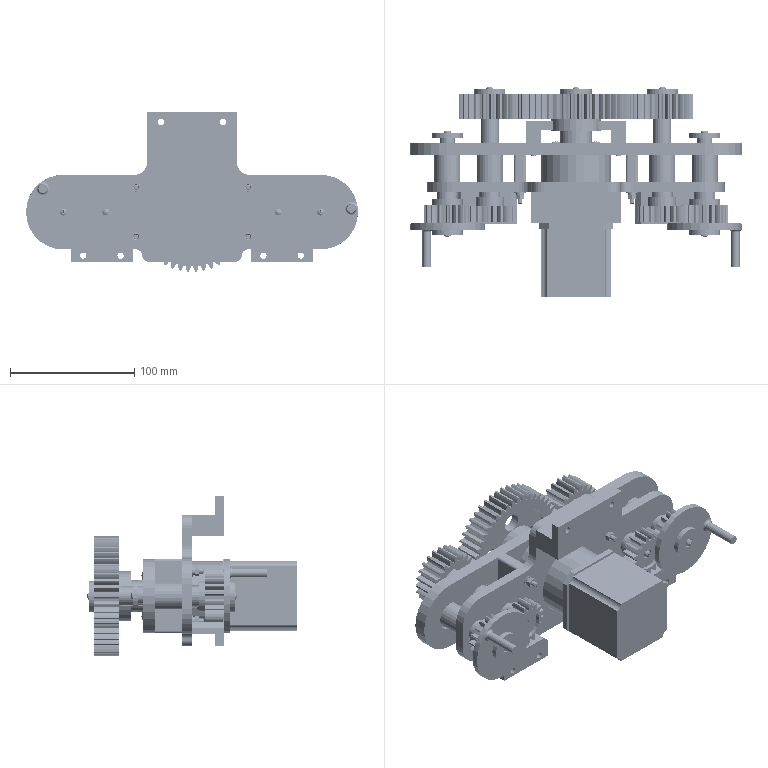Assembly | SolidWorks | mm | 113 component files | 113 solids | 4021 faces | box 266.76 x 168.69 x 128.09 mm | volume 977841 mm3 | cylinder 1324 | torus 964 | plane 785 | sphere 578 | cone 186 | spline 184 | commonest cylinder face diameters 13.6 x152 5 x65 4 x60 15 x54 87 x47 3 x46 96 x46 50 x46
Bill of materials:
23-ToothGear | 2 |  | Spur gear with straight teeth (roughly 24 teeth) and a central round bore with one rectangular keyway notch; a raised annular hub or boss sits on one face.
46-ToothGear | 1 |  | Spur gear with fine straight teeth (roughly 44 teeth), a central bore with a keyway notch, and four evenly spaced circular lightening or through holes around the bore; a short hub is visible on one face.
BearingHousing | 1 | A-Glass Fiber | Bracket with a central thick annular ring and two rectangular arms on opposite sides. Each arm steps down into an offset block, and each block has a small through hole running along the arm direction.
CrankshaftNo.1 | 2 | 5154-O, Bar (SS) | Stepped round shaft with several coaxial diameter sections. The largest section is near the middle, and both ends are smaller. One end section has a lengthwise keyway slot, and the end faces show small conical center holes.
Rolling bearings 61803 GB 276-94 | 4 |  | Ball-bearing-like ring set: thin flat outer ring and inner ring, with one row of spherical balls (about 30) in the annular gap; there are faint, irregular features near the inner ring that could be a cage or mesh artifacts.
Rolling bearings 61802 GB 276-94 | 4 |  | Ball-bearing-like ring set: flat outer and inner rings with one row of spherical balls (about 28) in the annular gap; open faces with no visible cage or shield.
NewCrank | 2 | AISI 1045 Steel, Cold Drawn | Flat circular disc with a central bore that has a keyway notch. A single cylindrical pin projects perpendicular to the disc face near the outer edge, with a fillet where it meets the disc.
GB - Spur gear 2M 17T 20PA 15FW ---S17B25H20L15.0S1 | 2 |  | Spur-gear-like body with about 17 straight teeth cut parallel to the axis, a round central bore with a rectangular keyway-like notch, and a smaller-diameter cylindrical hub boss on one face.
Rolling bearings 61804 GB 276-94 | 2 |  | Ball-bearing-like ring set: flat outer and inner rings with one row of spherical balls (about 28) in the annular gap; open faces with no visible cage or shield.
DialAxisNo.3 | 1 |  | Stepped cylindrical shaft/sleeve with a larger collar between two medium-diameter sections and a smaller-diameter spigot at one end. The larger end has an internal bore with a keyway notch, and the small spigot has an external lengthwise keyway slot.
EndCap4mm | 9 | 5454-O | Plain flat circular disc with a small central through hole and uniform thickness.
GB 93-87-3 | 9 |  | Split ring with a rectangular cross-section and a single narrow radial gap through the ring. It looks like a split or spring-type washer.
GB 93-87-4 | 10 |  | Split ring with a rectangular cross-section and a single narrow radial gap. It looks like a split or spring-type washer.
GB_T1096-1979PlainParallelKeyC-type5_12 | 2 |  | Rectangular-section bar with one end fully rounded and the other end square. All long edges are lightly rounded. It looks like a parallel key.
GB_T1096-1979PlainParallelKeyC-type5_18 | 3 |  | Rectangular-section bar with one rounded end and one square-cut end, and lightly rounded long edges. It looks like a parallel key.
GB_T1096-1979PlainParallelKeyC-type5_25 | 1 |  | Long rectangular-section bar with a rounded end visible at one end, a square-cut opposite end, and small edge rounds. It looks like a parallel key.
GB_T1096-1979PlainParallelKeyC-type5_25 | 2 |  | Straight bar with a near-square cross-section and rounded longitudinal edges. One end is flat and square-cut; the other end is fully rounded (semicircular) in one view. The shape looks like a parallel key.
GB_T6170-2000Type1HexNutGradeAAndBM4 | 4 |  | Hexagonal nut-like prism with a central through bore and chamfered corners on both faces.
GB_T818-2000PhillipsPanHeadScrewM3_12 | 9 |  | Fastener-like pin with a slotted domed head and a smooth cylindrical shank. The shank has a short reduced-diameter neck under the head and a chamfered tip.
GB_T818-2000PhillipsPanHeadScrewM4_12 | 4 |  | Slotted domed-head pin or screw-like part with a short smooth shank, a reduced neck under the head and a chamfered tip. Shorter and stubbier than similar parts in this set.
GB_T818-2000PhillipsPanHeadScrewM4_25 | 2 |  | Long, slender slotted domed-head pin or screw-like part with a smooth shank, a reduced neck under the head and a chamfered tip.
GB_T818-2000PhillipsPanHeadScrewM4_45 | 4 |  | Very long, slender slotted domed-head pin or screw-like part with a smooth shank, a small neck under the head and a chamfered tip.
GB_T95-2002FlatWasherCClass4x0.8 | 10 |  | Flat annular washer-like ring with a central circular hole and plain flat faces.
GB_T95-2002FlatWasherGradeC3_0.5 | 9 |  | Flat annular washer-like ring with a central circular hole. It looks slightly thinner than unnamed part.
GB823-88PhillipsSmallPanHeadScrewM5_14 | 2 |  | Short slotted domed-head pin or screw-like part. It has a relatively large head, a smooth shank, a reduced neck under the head and a chamfered tip.
GearIntermediateAxis | 2 | 5154-O, Bar (SS) | Stepped cylindrical shaft. It has a larger central collar, several smaller diameter steps toward each end, a keyway-like slot near each end and a small axial center hole in one end face.
GenevaWheelUpperGear(45Steel) | 2 |  | Spur-gear-like toothed wheel with a cylindrical hub on one side and a central bore with one rectangular keyway notch.
LatestLowerBaseFrame | 1 | 6061 Alloy | Thin flat plate with a cross or T-like outline and rounded corners. It has one large central hole, four medium round holes in line along the long axis, and several small holes.
LatestStepperMotor | 1 | AISI 1045 Steel, Cold Drawn | Simplified housing-like body. A square block with chamfered corners joins through a thin flange or collar to a cylindrical section, and a small stepped cylindrical shaft projects from the far end.
LegSupport | 2 |  | Prismatic block with an L-shaped cross-section (a full-width top portion over a narrower lower leg along one side), angled chamfers on the top edges at both short ends, and two round through holes in the long front face near each end.
LegSupport2 | 1 |  | Long rectangular bar with an L-shaped cross-section (a rabbet or step cut along one long top edge for the full length) and two round through holes in the large side face near the ends.
Support | 2 |  | Rectangular block or spacer bar with rounded long edges, and two round through holes passing through its narrow dimension near each end.
UpperBracket | 1 | 6061-T6 (SS) | Thin flat plate with a slot-shaped (obround) outline and fully rounded ends. It has a large central hole, four medium holes in line along the long axis (two near each end), and ten small holes grouped symmetrically around the center.
Mates:
1. concentric | LatestLowerBaseFrame-1 face at (-121.534, 78.266, -110.507) dir (0, 1, 0) r 2.5 | LegSupport2-1 face at (-121.534, 78.266, -110.507) dir (0, 1, 0) r 2.5
2. concentric | LatestLowerBaseFrame-1 face at (-71.534, 78.266, -110.507) dir (0, 1, 0) r 2.5 | LegSupport2-1 face at (-71.534, 78.266, -110.507) dir (0, 1, 0) r 2.5
3. coincident | LatestLowerBaseFrame-1 face at (-96.534, 78.266, -166.507) dir (0, -1, 0) | LegSupport2-1 face at (-96.534, 78.266, -102.347) dir (0, 1, 0)
4. concentric | LatestLowerBaseFrame-1 face at (-183.914, 78.265, -189.507) dir (0, 1, 0) r 1.6 | LegSupport-2 face at (-183.914, 78.266, -189.507) dir (0, 1, 0) r 1.25
5. concentric | LatestLowerBaseFrame-1 face at (-153.914, 78.265, -189.507) dir (0, 1, 0) r 1.6 | LegSupport-2 face at (-153.914, 78.266, -189.507) dir (0, 1, 0) r 1.25
6. coincident | LatestLowerBaseFrame-1 face at (-96.534, 78.266, -166.507) dir (0, -1, 0) | LegSupport-2 face at (-168.914, 78.266, -195.507) dir (0, 1, 0)
7. concentric | LatestLowerBaseFrame-1 face at (-9.154, 78.265, -189.507) dir (0, 1, 0) r 1.6 | LegSupport-1 face at (-9.154, 78.266, -189.507) dir (0, 1, 0) r 1.25
8. concentric | LatestLowerBaseFrame-1 face at (-39.154, 78.265, -189.507) dir (0, 1, 0) r 1.6 | LegSupport-1 face at (-39.154, 78.266, -189.507) dir (0, 1, 0) r 1.25
9. coincident | LatestLowerBaseFrame-1 face at (-96.534, 78.266, -166.507) dir (0, -1, 0) | LegSupport-1 face at (-24.154, 78.266, -195.507) dir (0, 1, 0)
10. concentric | CrankshaftOne-1/deep groove ball bearings gb-1 face at (-199.914, 75.055, -166.507) dir (0, -1, 0) r 13 | LatestLowerBaseFrame-1 face at (-199.914, 81.266, -166.507) dir (0, 1, 0) r 13
11. coincident | CrankshaftOne-1/deep groove ball bearings gb-1 face at (-207.438, 81.266, -173.095) dir (0, -1, 0) | LatestLowerBaseFrame-1 face at (-199.914, 81.266, -166.507) dir (0, 1, 0)
12. concentric | LatestLowerBaseFrame-1 face at (-51.534, 86.267, -146.507) dir (0, -1, 0) r 2 | Support-1 face at (-51.534, 108.266, -146.507) dir (0, -1, 0) r 2
13. concentric | LatestLowerBaseFrame-1 face at (-51.534, 86.267, -186.507) dir (0, -1, 0) r 2 | Support-1 face at (-51.534, 108.266, -186.507) dir (0, -1, 0) r 2
14. coincident | LatestLowerBaseFrame-1 face at (-96.534, 86.266, -166.507) dir (0, 1, 0) | Support-1 face at (-51.534, 86.266, -166.507) dir (0, -1, 0)
15. concentric | LatestLowerBaseFrame-1 face at (-141.534, 86.267, -186.507) dir (0, -1, 0) r 2 | Support-3 face at (-141.534, 108.266, -186.507) dir (0, -1, 0) r 2
16. concentric | LatestLowerBaseFrame-1 face at (-141.534, 86.267, -146.507) dir (0, -1, 0) r 2 | Support-3 face at (-141.534, 108.266, -146.507) dir (0, -1, 0) r 2
17. coincident | LatestLowerBaseFrame-1 face at (-96.534, 86.266, -166.507) dir (0, 1, 0) | Support-3 face at (-141.534, 86.266, -166.507) dir (0, -1, 0)
18. concentric | CrankshaftOne-2/deep groove ball bearings gb-1 face at (6.846, 75.055, -166.507) dir (0, -1, 0) r 13 | LatestLowerBaseFrame-1 face at (6.846, 81.266, -166.507) dir (0, 1, 0) r 13
19. coincident | CrankshaftOne-2/deep groove ball bearings gb-1 face at (5.649, 81.266, -156.579) dir (0, -1, 0) | LatestLowerBaseFrame-1 face at (6.846, 81.266, -166.507) dir (0, 1, 0)
20. concentric | LatestStepperMotor-1 face at (-96.534, 108.266, -166.507) dir (0, -1, 0) r 28 | LatestLowerBaseFrame-1 face at (-96.534, 78.266, -166.507) dir (0, 1, 0) r 28.5
21. concentric | DialAxis-1/DialAxisNo.3-1 face at (-96.534, 136.766, -166.507) dir (0, -1, 0) r 6 | LatestStepperMotor-1 face at (-96.534, 136.766, -166.507) dir (0, -1, 0) r 6
22. concentric | UpperBracket-2 face at (-141.534, 118.267, -186.507) dir (0, -1, 0) r 2 | Support-3 face at (-141.534, 108.266, -186.507) dir (0, -1, 0) r 2
23. concentric | UpperBracket-2 face at (-51.534, 118.267, -186.507) dir (0, -1, 0) r 2 | Support-1 face at (-51.534, 108.266, -186.507) dir (0, -1, 0) r 2
24. concentric | UpperBracket-2 face at (-80.624, 108.265, -182.417) dir (0, 1, 0) r 2.5 | LatestStepperMotor-1 face at (-80.624, 108.266, -182.417) dir (0, 1, 0) r 2.1
25. concentric | UpperBracket-2 face at (-112.444, 108.265, -150.597) dir (0, 1, 0) r 2.5 | LatestStepperMotor-1 face at (-112.444, 108.266, -150.597) dir (0, 1, 0) r 2.1
26. coincident | UpperBracket-2 face at (-96.534, 108.266, -166.507) dir (0, -1, 0) | Support-3 face at (-141.534, 108.266, -166.507) dir (0, 1, 0)
27. coincident | DialAxis-1/deep groove ball bearings gb-1 face at (-86.558, 111.266, -167.19) dir (0, -1, 0) | UpperBracket-2 face at (-96.534, 111.266, -166.507) dir (0, 1, 0)
28. concentric | UpperBracket-2 face at (-130.534, 108.265, -166.507) dir (0, 1, 0) r 2.5 | BearingHousing-2 face at (-130.534, 137.266, -166.507) dir (0, -1, 0) r 2.5
29. concentric | UpperBracket-2 face at (-62.534, 108.265, -166.507) dir (0, 1, 0) r 2.5 | BearingHousing-2 face at (-62.534, 137.266, -166.507) dir (0, -1, 0) r 2.5
30. concentric | DialAxis-1/deep groove ball bearings gb-2 face at (-96.534, 125.055, -166.507) dir (0, -1, 0) r 16 | BearingHousing-2 face at (-96.534, 130.266, -166.507) dir (0, 1, 0) r 16
31. coincident | UpperBracket-2 face at (-96.534, 118.266, -166.507) dir (0, 1, 0) | BearingHousing-2 face at (-96.534, 118.266, -166.507) dir (0, -1, 0)
32. concentric | DialAxis-1/DialAxisNo.3-1 face at (-96.534, 156.266, -166.507) dir (0, 1, 0) r 7.5 | 46-ToothGear-1 face at (-96.534, 137.266, -166.507) dir (0, 1, 0) r 7.5
33. coincident | DialAxis-1/DialAxisNo.3-1 face at (-89.034, 137.266, -166.507) dir (0, 1, 0) | 46-ToothGear-1 face at (-142.298, 137.266, -168.457) dir (0, -1, 0)
34. concentric | CrankshaftOne-1/CrankshaftNo.1-1 face at (-199.914, 122.266, -166.507) dir (0, 1, 0) r 1.65 | EndCap4mm-2 face at (-199.914, 124.266, -166.507) dir (0, 1, 0) r 4
35. concentric | CrankshaftOne-1/CrankshaftNo.1-1 face at (-199.914, 49.266, -166.507) dir (0, -1, 0) r 1.65 | EndCap4mm-4 face at (-199.914, 44.266, -166.507) dir (0, 1, 0) r 1.5
36. coincident | CrankshaftOne-1/CrankshaftNo.1-1 face at (-204.428, 122.266, -170.46) dir (0, 1, 0) | EndCap4mm-2 face at (-199.914, 122.266, -166.507) dir (0, -1, 0)
37. coincident | CrankshaftOne-2/CrankshaftNo.1-1 face at (6.128, 122.266, -160.55) dir (0, 1, 0) | EndCap4mm-1 face at (6.846, 122.266, -166.507) dir (0, -1, 0)
38. concentric | CrankshaftOne-2/CrankshaftNo.1-1 face at (6.846, 122.266, -166.507) dir (0, 1, 0) r 1.65 | EndCap4mm-1 face at (6.846, 124.266, -166.507) dir (0, 1, 0) r 4
39. coincident | CrankshaftOne-1/NewCrank-1 face at (-199.914, 48.266, -166.507) dir (0, -1, 0) | EndCap4mm-4 face at (-199.914, 48.266, -166.507) dir (0, 1, 0)
40. coincident | CrankshaftOne-2/NewCrank-1 face at (6.846, 48.266, -166.507) dir (0, -1, 0) | EndCap4mm-3 face at (6.846, 48.266, -166.507) dir (0, 1, 0)
41. concentric | CrankshaftOne-2/CrankshaftNo.1-1 face at (6.846, 49.266, -166.507) dir (0, -1, 0) r 1.65 | EndCap4mm-3 face at (6.846, 44.266, -166.507) dir (0, 1, 0) r 1.5
42. coincident | 23-ToothGear-2 face at (-27.344, 157.266, -166.507) dir (0, 1, 0) | EndCap4mm-6 face at (-27.344, 157.266, -166.507) dir (0, -1, 0)
43. coincident | 23-ToothGear-1 face at (-165.724, 157.266, -166.507) dir (0, 1, 0) | EndCap4mm-5 face at (-165.724, 157.266, -166.507) dir (0, -1, 0)
44. coincident | DialAxis-1/DialAxisNo.3-1 face at (-94.034, 156.266, -152.007) dir (-1, 0, 0) | 46-ToothGear-1 face at (-94.034, 137.265, -166.507) dir (-1, 0, 0)
45. coincident | DialAxis-1/DialAxisNo.3-1 face at (-99.034, 156.266, -152.007) dir (1, 0, 0) | 46-ToothGear-1 face at (-99.034, 137.265, -166.507) dir (1, 0, 0)
46. coincident | GenevaWheelUpperGear(45Steel)-2 face at (-165.724, 61.266, -166.507) dir (0, -1, 0) | EndCap4mm-7 face at (-165.724, 61.266, -166.507) dir (0, 1, 0)
47. coincident | GenevaWheelUpperGear(45Steel)-1 face at (-27.344, 61.266, -166.507) dir (0, -1, 0) | EndCap4mm-8 face at (-27.344, 61.266, -166.507) dir (0, 1, 0)
48. concentric | DialAxis-1/DialAxisNo.3-1 face at (-96.534, 156.266, -166.507) dir (0, 1, 0) r 1.5 | EndCap4mm-9 face at (-96.534, 161.266, -166.507) dir (0, -1, 0) r 1.5
49. coincident | 46-ToothGear-1 face at (-96.534, 157.266, -166.507) dir (0, 1, 0) | EndCap4mm-9 face at (-96.534, 157.266, -166.507) dir (0, -1, 0)
50. coincident | LatestLowerBaseFrame-1 face at (-165.724, 81.266, -166.507) dir (0, 1, 0) | deep groove ball bearings gb-1 face at (-174.739, 81.266, -170.835) dir (0, -1, 0)
51. concentric | LatestLowerBaseFrame-1 face at (-165.724, 81.266, -166.507) dir (0, 1, 0) r 13 | deep groove ball bearings gb-1 face at (-165.724, 75.055, -166.507) dir (0, -1, 0) r 13
52. coincident | LatestLowerBaseFrame-1 face at (-27.344, 81.266, -166.507) dir (0, 1, 0) | deep groove ball bearings gb-2 face at (-36.359, 81.266, -170.835) dir (0, -1, 0)
53. concentric | LatestLowerBaseFrame-1 face at (-27.344, 81.266, -166.507) dir (0, 1, 0) r 13 | deep groove ball bearings gb-2 face at (-27.344, 75.055, -166.507) dir (0, -1, 0) r 13
54. coincident | UpperBracket-2 face at (-165.724, 116.266, -166.507) dir (0, -1, 0) | deep groove ball bearings gb-3 face at (-172.485, 116.266, -169.753) dir (0, 1, 0)
55. concentric | UpperBracket-2 face at (-165.724, 116.266, -166.507) dir (0, -1, 0) r 12 | deep groove ball bearings gb-3 face at (-165.724, 105.055, -166.507) dir (0, -1, 0) r 12
56. coincident | UpperBracket-2 face at (-27.344, 116.266, -166.507) dir (0, -1, 0) | deep groove ball bearings gb-4 face at (-34.105, 116.266, -169.753) dir (0, 1, 0)
57. concentric | UpperBracket-2 face at (-27.344, 116.266, -166.507) dir (0, -1, 0) r 12 | deep groove ball bearings gb-4 face at (-27.344, 105.055, -166.507) dir (0, -1, 0) r 12
58. concentric | deep groove ball bearings gb-1 face at (-165.724, 76.795, -166.507) dir (0, -1, 0) r 8.5 | GearIntermediateAxis-1 face at (-165.724, 172.745, -166.507) dir (0, 1, 0) r 10.5
59. coincident | deep groove ball bearings gb-1 face at (-173.387, 86.266, -170.186) dir (0, 1, 0) | GearIntermediateAxis-1 face at (-170.562, 86.266, -157.188) dir (0, -1, 0)
60. concentric | 23-ToothGear-1 face at (-165.724, 157.266, -166.507) dir (0, -1, 0) r 6 | GearIntermediateAxis-1 face at (-165.724, 172.745, -166.507) dir (0, 1, 0) r 6
61. coincident | 23-ToothGear-1 face at (-177.832, 137.266, -147.143) dir (0, -1, 0) | GearIntermediateAxis-1 face at (-168.488, 137.266, -161.182) dir (0, 1, 0)
62. coincident | GenevaWheelUpperGear(45Steel)-2 face at (-165.724, 74.266, -166.507) dir (0, 1, 0) | GearIntermediateAxis-1 face at (-169.64, 74.266, -158.963) dir (0, -1, 0)
63. concentric | deep groove ball bearings gb-2 face at (-27.344, 76.795, -166.507) dir (0, -1, 0) r 8.5 | GearIntermediateAxis-2 face at (-27.344, 172.745, -166.507) dir (0, 1, 0) r 10.5
64. coincident | GearIntermediateAxis-1 face at (-165.724, 157.266, -166.507) dir (0, 1, 0) | GearIntermediateAxis-2 face at (-27.344, 157.266, -166.507) dir (0, 1, 0)
65. concentric | 23-ToothGear-2 face at (-27.344, 157.266, -166.507) dir (0, -1, 0) r 6 | GearIntermediateAxis-2 face at (-27.344, 172.745, -166.507) dir (0, 1, 0) r 6
66. coincident | GenevaWheelUpperGear(45Steel)-1 face at (-27.344, 74.266, -166.507) dir (0, 1, 0) | GearIntermediateAxis-2 face at (-27.924, 74.266, -158.027) dir (0, -1, 0)
67. coincident | 23-ToothGear-2 face at (-30.717, 137.266, -143.92) dir (0, -1, 0) | GearIntermediateAxis-2 face at (-27.753, 137.266, -160.521) dir (0, 1, 0)
68. concentric | GenevaWheelUpperGear(45Steel)-2 face at (-165.724, 54.266, -166.507) dir (0, 1, 0) r 7.5 | GearIntermediateAxis-1 face at (-165.724, 172.745, -166.507) dir (0, 1, 0) r 7.5
69. coincident | GenevaWheelUpperGear(45Steel)-1 face at (-27.344, 74.266, -166.507) dir (0, 1, 0) | GearIntermediateAxis-2 face at (-27.924, 74.266, -158.027) dir (0, -1, 0)
70. concentric | GenevaWheelUpperGear(45Steel)-1 face at (-27.344, 54.266, -166.507) dir (0, 1, 0) r 7.5 | GearIntermediateAxis-2 face at (-27.344, 172.745, -166.507) dir (0, 1, 0) r 7.5
71. concentric | GearIntermediateAxis-1 face at (-161.73, 70.766, -164.434) dir (0.8876, 0, 0.4607) r 2.5 | GB_T1096-1979PlainParallelKeyC-type5_12-1 face at (-161.73, 70.766, -164.434) dir (0.8876, 0, 0.4607) r 2.5
72. coincident | GearIntermediateAxis-1 face at (-160.579, 61.266, -166.653) dir (-0.4607, 0, 0.8876) | GB_T1096-1979PlainParallelKeyC-type5_12-1 face at (-160.579, 70.766, -166.653) dir (0.4607, 0, -0.8876)
73. coincident | GearIntermediateAxis-1 face at (-161.73, 61.266, -164.434) dir (0.8876, 0, 0.4607) | GB_T1096-1979PlainParallelKeyC-type5_12-1 face at (-161.73, 70.766, -164.434) dir (-0.8876, 0, -0.4607)
74. coincident | GenevaWheelUpperGear(45Steel)-2 face at (-158, 54.266, -159.681) dir (0.4607, 0, -0.8876) | GB_T1096-1979PlainParallelKeyC-type5_12-1 face at (-162.882, 70.766, -162.215) dir (-0.4607, 0, 0.8876)
75. concentric | GB_T1096-1979PlainParallelKeyC-type5_18-1 face at (-158.624, 141.766, -162.822) dir (-0.8876, 0, -0.4607) r 2.5 | GearIntermediateAxis-1 face at (-163.062, 141.766, -165.125) dir (0.8876, 0, 0.4607) r 2.5
76. coincident | GearIntermediateAxis-1 face at (-164.213, 157.266, -162.906) dir (0.4607, 0, -0.8876) | GB_T1096-1979PlainParallelKeyC-type5_18-1 face at (-159.776, 141.766, -160.603) dir (-0.4607, 0, 0.8876)
77. coincident | GearIntermediateAxis-1 face at (-163.062, 157.266, -165.125) dir (0.8876, 0, 0.4607) | GB_T1096-1979PlainParallelKeyC-type5_18-1 face at (-163.062, 141.766, -165.125) dir (-0.8876, 0, -0.4607)
78. coincident | 23-ToothGear-1 face at (-164.573, 157.267, -168.726) dir (-0.4607, 0, 0.8876) | GB_T1096-1979PlainParallelKeyC-type5_18-1 face at (-157.472, 141.766, -165.041) dir (0.4607, 0, -0.8876)
79. concentric | GearIntermediateAxis-2 face at (-24.351, 141.766, -166.303) dir (0.9977, 0, 0.06814) r 2.5 | GB_T1096-1979PlainParallelKeyC-type5_18-2 face at (-19.363, 141.766, -165.962) dir (-0.9977, 0, -0.06814) r 2.5
80. coincident | GearIntermediateAxis-2 face at (-24.351, 157.266, -166.303) dir (0.9977, 0, 0.06814) | GB_T1096-1979PlainParallelKeyC-type5_18-2 face at (-24.351, 141.766, -166.303) dir (-0.9977, 0, -0.06814)
81. coincident | 23-ToothGear-2 face at (-27.174, 157.267, -169.001) dir (-0.06814, 0, 0.9977) | GB_T1096-1979PlainParallelKeyC-type5_18-2 face at (-19.193, 141.766, -168.456) dir (0.06814, 0, -0.9977)
82. concentric | GearIntermediateAxis-2 face at (-22.855, 70.766, -166.2) dir (0.9977, 0, 0.06814) r 2.5 | GB_T1096-1979PlainParallelKeyC-type5_12-2 face at (-22.855, 70.766, -166.2) dir (0.9977, 0, 0.06814) r 2.5
83. coincident | GearIntermediateAxis-2 face at (-22.855, 61.266, -166.2) dir (0.9977, 0, 0.06814) | GB_T1096-1979PlainParallelKeyC-type5_12-2 face at (-22.855, 70.766, -166.2) dir (-0.9977, 0, -0.06814)
84. coincident | GenevaWheelUpperGear(45Steel)-1 face at (-17.538, 54.266, -163.332) dir (0.06814, 0, -0.9977) | GB_T1096-1979PlainParallelKeyC-type5_12-2 face at (-23.025, 70.766, -163.706) dir (-0.06814, 0, 0.9977)
85. coincident | 23-ToothGear-2 face at (-27.344, 157.266, -166.507) dir (0, 1, 0) | EndCap4mm-6 face at (-27.344, 157.266, -166.507) dir (0, -1, 0)
86. concentric | EndCap4mm-6 face at (-27.344, 161.266, -166.507) dir (0, -1, 0) r 1.5 | GearIntermediateAxis-2 face at (-27.344, 157.266, -166.507) dir (0, 1, 0) r 1.5
87. coincident | 23-ToothGear-1 face at (-165.724, 157.266, -166.507) dir (0, 1, 0) | EndCap4mm-5 face at (-165.724, 157.266, -166.507) dir (0, -1, 0)
88. concentric | EndCap4mm-5 face at (-165.724, 161.266, -166.507) dir (0, -1, 0) r 1.5 | GearIntermediateAxis-1 face at (-165.724, 157.266, -166.507) dir (0, 1, 0) r 1.5
89. coincident | GenevaWheelUpperGear(45Steel)-2 face at (-165.724, 61.266, -166.507) dir (0, -1, 0) | EndCap4mm-7 face at (-165.724, 61.266, -166.507) dir (0, 1, 0)
90. concentric | EndCap4mm-7 face at (-165.724, 57.266, -166.507) dir (0, 1, 0) r 1.5 | GearIntermediateAxis-1 face at (-165.724, 61.266, -166.507) dir (0, -1, 0) r 1.5
91. coincident | GenevaWheelUpperGear(45Steel)-1 face at (-27.344, 61.266, -166.507) dir (0, -1, 0) | EndCap4mm-8 face at (-27.344, 61.266, -166.507) dir (0, 1, 0)
92. concentric | EndCap4mm-8 face at (-27.344, 57.266, -166.507) dir (0, 1, 0) r 1.5 | GearIntermediateAxis-2 face at (-27.344, 61.266, -166.507) dir (0, -1, 0) r 1.5
93. concentric | DialAxis-1/DialAxisNo.3-1 face at (-96.534, 140.766, -152.007) dir (0, 0, -1) r 2.5 | GB_T1096-1979PlainParallelKeyC-type5_18-3 face at (-96.534, 140.766, -162.007) dir (0, 0, 1) r 2.5
94. coincident | DialAxis-1/DialAxisNo.3-1 face at (-96.534, 156.266, -162.007) dir (0, 0, 1) | GB_T1096-1979PlainParallelKeyC-type5_18-3 face at (-96.534, 140.766, -162.007) dir (0, 0, -1)
95. coincident | DialAxis-1/DialAxisNo.3-1 face at (-94.034, 136.766, -166.507) dir (-1, 0, 0) | LatestStepperMotor-1 face at (-94.034, 136.766, -169.507) dir (-1, 0, 0)
96. concentric | LatestStepperMotor-1 face at (-96.534, 114.266, -169.507) dir (0, 0, -1) r 2.5 | GB_T1096-1979PlainParallelKeyC-type5_25-1 face at (-96.534, 114.266, -169.507) dir (0, 0, -1) r 2.5
97. coincident | LatestStepperMotor-1 face at (-99.034, 136.766, -169.507) dir (1, 0, 0) | GB_T1096-1979PlainParallelKeyC-type5_25-1 face at (-99.034, 114.266, -169.507) dir (-1, 0, 0)
98. coincident | LatestStepperMotor-1 face at (-96.534, 136.766, -169.507) dir (0, 0, -1) | GB_T1096-1979PlainParallelKeyC-type5_25-1 face at (-96.534, 114.266, -169.507) dir (0, 0, 1)
99. coincident | UpperBracket-2 face at (-96.534, 108.266, -166.507) dir (0, -1, 0) | LatestStepperMotor-1 face at (-96.534, 108.266, -166.507) dir (0, 1, 0)
100. concentric | CrankshaftOne-2/CrankshaftNo.1-1 face at (2.378, 68.766, -167.046) dir (-0.9928, 0, -0.1196) r 2.5 | GB_T1096-1979PlainParallelKeyC-type5_25-2 face at (2.378, 68.766, -167.046) dir (-0.9928, 0, -0.1196) r 2.5
101. coincident | CrankshaftOne-2/CrankshaftNo.1-1 face at (2.378, 68.766, -167.046) dir (-0.9928, 0, -0.1196) | GB_T1096-1979PlainParallelKeyC-type5_25-2 face at (2.378, 68.766, -167.046) dir (0.9928, 0, 0.1196)
102. coincident | CrankshaftOne-2/CrankshaftNo.1-1 face at (2.079, 68.766, -164.563) dir (0.1196, 0, -0.9928) | GB_T1096-1979PlainParallelKeyC-type5_25-2 face at (2.079, 68.766, -164.563) dir (-0.1196, 0, 0.9928)
103. concentric | CrankshaftOne-1/CrankshaftNo.1-1 face at (-196.95, 68.766, -169.893) dir (0.6588, 0, -0.7523) r 2.5 | GB_T1096-1979PlainParallelKeyC-type5_25-3 face at (-196.95, 68.766, -169.893) dir (0.6588, 0, -0.7523) r 2.5
104. coincident | CrankshaftOne-1/CrankshaftNo.1-1 face at (-196.95, 68.766, -169.893) dir (0.6588, 0, -0.7523) | GB_T1096-1979PlainParallelKeyC-type5_25-3 face at (-196.95, 68.766, -169.893) dir (-0.6588, 0, 0.7523)
105. coincident | CrankshaftOne-1/CrankshaftNo.1-1 face at (-198.831, 68.766, -171.54) dir (0.7523, 0, 0.6588) | GB_T1096-1979PlainParallelKeyC-type5_25-3 face at (-198.831, 68.766, -171.54) dir (-0.7523, 0, -0.6588)
106. coincident | EndCap4mm-9 face at (-96.534, 159.266, -166.507) dir (0, 1, 0) | GB_T95-2002FlatWasherGradeC3_0.5-1 face at (-95.111, 159.266, -165.577) dir (0, -1, 0)
107. concentric | EndCap4mm-9 face at (-96.534, 161.266, -166.507) dir (0, -1, 0) r 1.5 | GB_T95-2002FlatWasherGradeC3_0.5-1 face at (-96.534, 168.41, -166.507) dir (0, 1, 0) r 1.7
108. concentric | EndCap4mm-9 face at (-96.534, 161.266, -166.507) dir (0, -1, 0) r 1.5 | GB 93-87-3-1 face at (-96.534, 160.566, -166.507) dir (0, -1, 0) r 1.55
109. coincident | GB 93-87-3-1 face at (-96.534, 159.766, -166.507) dir (0, -1, 0) | GB_T95-2002FlatWasherGradeC3_0.5-1 face at (-95.111, 159.766, -165.577) dir (0, 1, 0)
110. concentric | EndCap4mm-9 face at (-96.534, 161.266, -166.507) dir (0, -1, 0) r 1.5 | GB_T818-2000PhillipsPanHeadScrewM3_12-1 face at (-96.534, 164.298, -166.507) dir (0, 1, 0) r 1.5
111. coincident | GB 93-87-3-1 face at (-96.534, 160.566, -166.507) dir (0, 1, 0) | GB_T818-2000PhillipsPanHeadScrewM3_12-1 face at (-95.034, 160.566, -166.507) dir (0, -1, 0)
112. coincident | EndCap4mm-5 face at (-165.724, 159.266, -166.507) dir (0, 1, 0) | GB_T95-2002FlatWasherGradeC3_0.5-2 face at (-166.76, 159.266, -167.855) dir (0, -1, 0)
113. concentric | EndCap4mm-5 face at (-165.724, 161.266, -166.507) dir (0, -1, 0) r 1.5 | GB_T95-2002FlatWasherGradeC3_0.5-2 face at (-165.724, 168.41, -166.507) dir (0, 1, 0) r 1.7
114. coincident | GB_T95-2002FlatWasherGradeC3_0.5-2 face at (-166.76, 159.766, -167.855) dir (0, 1, 0) | GB 93-87-3-4 face at (-165.724, 159.766, -166.507) dir (0, -1, 0)
115. concentric | EndCap4mm-5 face at (-165.724, 161.266, -166.507) dir (0, -1, 0) r 1.5 | GB 93-87-3-4 face at (-165.724, 160.566, -166.507) dir (0, -1, 0) r 1.55
116. concentric | EndCap4mm-5 face at (-165.724, 161.266, -166.507) dir (0, -1, 0) r 1.5 | GB_T818-2000PhillipsPanHeadScrewM3_12-2 face at (-165.724, 164.298, -166.507) dir (0, 1, 0) r 1.5
117. coincident | GB_T818-2000PhillipsPanHeadScrewM3_12-2 face at (-164.224, 160.566, -166.507) dir (0, -1, 0) | GB 93-87-3-4 face at (-165.724, 160.566, -166.507) dir (0, 1, 0)
118. coincident | EndCap4mm-6 face at (-27.344, 159.266, -166.507) dir (0, 1, 0) | GB_T95-2002FlatWasherGradeC3_0.5-3 face at (-25.921, 159.266, -165.577) dir (0, -1, 0)
119. concentric | EndCap4mm-6 face at (-27.344, 161.266, -166.507) dir (0, -1, 0) r 1.5 | GB_T95-2002FlatWasherGradeC3_0.5-3 face at (-27.344, 168.41, -166.507) dir (0, 1, 0) r 1.7
120. coincident | GB 93-87-3-5 face at (-27.344, 159.766, -166.507) dir (0, -1, 0) | GB_T95-2002FlatWasherGradeC3_0.5-3 face at (-25.921, 159.766, -165.577) dir (0, 1, 0)
121. concentric | EndCap4mm-6 face at (-27.344, 161.266, -166.507) dir (0, -1, 0) r 1.5 | GB 93-87-3-5 face at (-27.344, 160.566, -166.507) dir (0, -1, 0) r 1.55
122. concentric | EndCap4mm-6 face at (-27.344, 161.266, -166.507) dir (0, -1, 0) r 1.5 | GB_T818-2000PhillipsPanHeadScrewM3_12-3 face at (-27.344, 164.298, -166.507) dir (0, 1, 0) r 1.5
123. coincident | GB_T818-2000PhillipsPanHeadScrewM3_12-3 face at (-25.844, 160.566, -166.507) dir (0, -1, 0) | GB 93-87-3-5 face at (-27.344, 160.566, -166.507) dir (0, 1, 0)
124. coincident | BearingHousing-2 face at (-130.534, 130.266, -166.507) dir (0, 1, 0) | GB_T95-2002FlatWasherCClass4x0.8-1 face at (-132.784, 130.266, -166.507) dir (0, -1, 0)
125. concentric | BearingHousing-2 face at (-130.534, 137.266, -166.507) dir (0, -1, 0) r 2.5 | GB_T95-2002FlatWasherCClass4x0.8-1 face at (-130.534, 121.621, -166.507) dir (0, -1, 0) r 2.25
126. coincident | GB 93-87-4-1 face at (-130.534, 131.066, -166.507) dir (0, -1, 0) | GB_T95-2002FlatWasherCClass4x0.8-1 face at (-132.784, 131.066, -166.507) dir (0, 1, 0)
127. concentric | BearingHousing-2 face at (-130.534, 137.266, -166.507) dir (0, -1, 0) r 2.5 | GB 93-87-4-1 face at (-130.534, 132.166, -166.507) dir (0, -1, 0) r 2.05
128. concentric | BearingHousing-2 face at (-130.534, 137.266, -166.507) dir (0, -1, 0) r 2.5 | GB_T818-2000PhillipsPanHeadScrewM4_25-1 face at (-130.534, 136.598, -166.507) dir (0, 1, 0) r 2
129. coincident | GB 93-87-4-1 face at (-130.534, 132.166, -166.507) dir (0, 1, 0) | GB_T818-2000PhillipsPanHeadScrewM4_25-1 face at (-128.584, 132.166, -166.507) dir (0, -1, 0)
130. coincident | BearingHousing-2 face at (-62.534, 130.266, -166.507) dir (0, 1, 0) | GB_T95-2002FlatWasherCClass4x0.8-2 face at (-64.784, 130.266, -166.507) dir (0, -1, 0)
131. concentric | BearingHousing-2 face at (-62.534, 137.266, -166.507) dir (0, -1, 0) r 2.5 | GB_T95-2002FlatWasherCClass4x0.8-2 face at (-62.534, 121.621, -166.507) dir (0, -1, 0) r 2.25
132. coincident | GB 93-87-4-2 face at (-62.534, 131.066, -166.507) dir (0, -1, 0) | GB_T95-2002FlatWasherCClass4x0.8-2 face at (-64.784, 131.066, -166.507) dir (0, 1, 0)
133. concentric | BearingHousing-2 face at (-62.534, 137.266, -166.507) dir (0, -1, 0) r 2.5 | GB 93-87-4-2 face at (-62.534, 132.166, -166.507) dir (0, -1, 0) r 2.05
134. concentric | BearingHousing-2 face at (-62.534, 137.266, -166.507) dir (0, -1, 0) r 2.5 | GB_T818-2000PhillipsPanHeadScrewM4_25-2 face at (-62.534, 136.598, -166.507) dir (0, 1, 0) r 2
135. coincident | GB 93-87-4-2 face at (-62.534, 132.166, -166.507) dir (0, 1, 0) | GB_T818-2000PhillipsPanHeadScrewM4_25-2 face at (-60.584, 132.166, -166.507) dir (0, -1, 0)
136. coincident | UpperBracket-2 face at (-112.444, 114.266, -150.597) dir (0, 1, 0) | GB_T95-2002FlatWasherCClass4x0.8-3 face at (-114.694, 114.266, -150.597) dir (0, -1, 0)
137. concentric | UpperBracket-2 face at (-112.444, 114.266, -150.597) dir (0, 1, 0) r 5 | GB_T95-2002FlatWasherCClass4x0.8-3 face at (-112.444, 105.621, -150.597) dir (0, -1, 0) r 2.25
138. coincident | GB_T95-2002FlatWasherCClass4x0.8-3 face at (-114.694, 115.066, -150.597) dir (0, 1, 0) | GB 93-87-4-3 face at (-112.444, 115.066, -150.597) dir (0, -1, 0)
139. concentric | UpperBracket-2 face at (-112.444, 114.266, -150.597) dir (0, 1, 0) r 5 | GB 93-87-4-3 face at (-112.444, 116.166, -150.597) dir (0, -1, 0) r 2.05
140. concentric | UpperBracket-2 face at (-112.444, 108.265, -150.597) dir (0, 1, 0) r 2.5 | GB_T818-2000PhillipsPanHeadScrewM4_12-1 face at (-112.444, 120.598, -150.597) dir (0, 1, 0) r 2
141. coincident | GB 93-87-4-3 face at (-112.444, 116.166, -150.597) dir (0, 1, 0) | GB_T818-2000PhillipsPanHeadScrewM4_12-1 face at (-110.494, 116.166, -150.597) dir (0, -1, 0)
142. coincident | UpperBracket-2 face at (-141.534, 114.266, -146.507) dir (0, 1, 0) | GB_T818-2000PhillipsPanHeadScrewM4_45-1 face at (-139.584, 114.266, -146.507) dir (0, -1, 0)
143. concentric | UpperBracket-2 face at (-141.534, 118.267, -146.507) dir (0, -1, 0) r 2 | GB_T818-2000PhillipsPanHeadScrewM4_45-1 face at (-141.534, 118.698, -146.507) dir (0, 1, 0) r 2
144. concentric | GB_T95-2002FlatWasherCClass4x0.8-7 face at (-141.534, 68.821, -146.507) dir (0, -1, 0) r 2.25 | GB_T818-2000PhillipsPanHeadScrewM4_45-1 face at (-141.534, 118.698, -146.507) dir (0, 1, 0) r 2
145. coincident | LatestLowerBaseFrame-1 face at (-96.534, 78.266, -166.507) dir (0, -1, 0) | GB_T95-2002FlatWasherCClass4x0.8-7 face at (-143.784, 78.266, -146.507) dir (0, 1, 0)
146. concentric | GB_T818-2000PhillipsPanHeadScrewM4_45-1 face at (-141.534, 118.698, -146.507) dir (0, 1, 0) r 2 | GB 93-87-4-7 face at (-141.534, 77.466, -146.507) dir (0, -1, 0) r 2.05
147. coincident | GB 93-87-4-7 face at (-141.534, 77.466, -146.507) dir (0, 1, 0) | GB_T95-2002FlatWasherCClass4x0.8-7 face at (-143.784, 77.466, -146.507) dir (0, -1, 0)
148. coincident | GB 93-87-4-7 face at (-141.534, 76.366, -146.507) dir (0, -1, 0) | GB_T6170-2000Type1HexNutGradeAAndBM4-1 face at (-134.901, 76.366, -146.481) dir (0, 1, 0)
149. concentric | GB_T818-2000PhillipsPanHeadScrewM4_45-1 face at (-141.534, 118.698, -146.507) dir (0, 1, 0) r 2 | GB_T6170-2000Type1HexNutGradeAAndBM4-1 face at (-141.534, 76.366, -146.507) dir (0, -1, 0) r 2
150. concentric | LegSupport2-1 face at (-121.534, 78.266, -110.507) dir (0, 1, 0) r 2.5 | GB823-88PhillipsSmallPanHeadScrewM5_14-1 face at (-121.534, 86.153, -110.507) dir (0, 1, 0) r 2.5
151. coincident | LatestLowerBaseFrame-1 edge at (-121.534, 82.266, -110.507) dir (0, 1, 0) r 5 | GB823-88PhillipsSmallPanHeadScrewM5_14-1 face at (-121.127, 82.266, -108.381) dir (0, -1, 0)
152. concentric | LegSupport2-1 face at (-71.534, 78.266, -110.507) dir (0, 1, 0) r 2.5 | GB823-88PhillipsSmallPanHeadScrewM5_14-2 face at (-71.534, 86.153, -110.507) dir (0, 1, 0) r 2.5
153. coincident | LatestLowerBaseFrame-1 face at (-71.534, 82.266, -110.507) dir (0, 1, 0) | GB823-88PhillipsSmallPanHeadScrewM5_14-2 face at (-71.127, 82.266, -108.381) dir (0, -1, 0)
154. coincident | EndCap4mm-2 face at (-199.914, 124.266, -166.507) dir (0, 1, 0) | GB_T95-2002FlatWasherGradeC3_0.5-7 face at (-200.95, 124.266, -167.855) dir (0, -1, 0)
155. concentric | EndCap4mm-2 face at (-199.914, 126.266, -166.507) dir (0, -1, 0) r 1.5 | GB_T95-2002FlatWasherGradeC3_0.5-7 face at (-199.914, 133.41, -166.507) dir (0, 1, 0) r 1.7
156. coincident | GB 93-87-3-8 face at (-199.914, 124.766, -166.507) dir (0, -1, 0) | GB_T95-2002FlatWasherGradeC3_0.5-7 face at (-200.95, 124.766, -167.855) dir (0, 1, 0)
157. concentric | EndCap4mm-2 face at (-199.914, 126.266, -166.507) dir (0, -1, 0) r 1.5 | GB 93-87-3-8 face at (-199.914, 125.566, -166.507) dir (0, -1, 0) r 1.55
158. concentric | EndCap4mm-2 face at (-199.914, 126.266, -166.507) dir (0, -1, 0) r 1.5 | GB_T818-2000PhillipsPanHeadScrewM3_12-6 face at (-199.914, 129.298, -166.507) dir (0, 1, 0) r 1.5
159. coincident | GB_T818-2000PhillipsPanHeadScrewM3_12-6 face at (-198.414, 125.566, -166.507) dir (0, -1, 0) | GB 93-87-3-8 face at (-199.914, 125.566, -166.507) dir (0, 1, 0)
160. coincident | EndCap4mm-1 face at (6.846, 124.266, -166.507) dir (0, 1, 0) | GB_T95-2002FlatWasherGradeC3_0.5-6 face at (8.45, 124.266, -167.069) dir (0, -1, 0)
161. concentric | EndCap4mm-1 face at (6.846, 126.266, -166.507) dir (0, -1, 0) r 1.5 | GB_T95-2002FlatWasherGradeC3_0.5-6 face at (6.846, 115.621, -166.507) dir (0, -1, 0) r 1.7
162. coincident | GB_T95-2002FlatWasherGradeC3_0.5-6 face at (8.45, 124.766, -167.069) dir (0, 1, 0) | GB 93-87-3-9 face at (6.846, 124.766, -166.507) dir (0, -1, 0)
163. concentric | EndCap4mm-1 face at (6.846, 126.266, -166.507) dir (0, -1, 0) r 1.5 | GB 93-87-3-9 face at (6.846, 125.566, -166.507) dir (0, -1, 0) r 1.55
164. concentric | EndCap4mm-1 face at (6.846, 126.266, -166.507) dir (0, -1, 0) r 1.5 | GB_T818-2000PhillipsPanHeadScrewM3_12-7 face at (6.846, 129.298, -166.507) dir (0, 1, 0) r 1.5
165. coincident | GB 93-87-3-9 face at (6.846, 125.566, -166.507) dir (0, 1, 0) | GB_T818-2000PhillipsPanHeadScrewM3_12-7 face at (8.346, 125.566, -166.507) dir (0, -1, 0)
166. concentric | CrankshaftNo.1-1 face at (-58.793, 6.699, 73) dir (-1, 0, 0) r 8.5 | deep groove ball bearings gb-1 face at (-31.264, 6.699, 73) dir (-1, 0, 0) r 8.5
167. coincident | CrankshaftNo.1-1 face at (-21.793, 15.199, 73) dir (-1, 0, 0) | deep groove ball bearings gb-1 face at (-21.793, 19.699, 73) dir (1, 0, 0)
168. concentric | CrankshaftNo.1-1 face at (-58.793, 6.699, 73) dir (-1, 0, 0) r 7.5 | deep groove ball bearings gb-2 face at (-1.264, 6.699, 73) dir (-1, 0, 0) r 7.5
169. coincident | CrankshaftNo.1-1 face at (3.207, 17.199, 73) dir (1, 0, 0) | deep groove ball bearings gb-2 face at (3.207, 18.699, 73) dir (-1, 0, 0)
170. concentric | CrankshaftNo.1-1 face at (-58.793, 6.699, 73) dir (-1, 0, 0) r 7.5 | spur gear_gb-1 face at (-59.793, 6.699, 73) dir (1, 0, 0) r 7.5
171. coincident | CrankshaftNo.1-1 face at (-34.793, 14.199, 73) dir (-1, 0, 0) | spur gear_gb-1 face at (-34.793, 6.699, 73) dir (1, 0, 0)
172. coincident | CrankshaftNo.1-1 face at (-61.085, 4.199, 68.5) dir (0, 1, 0) | spur gear_gb-1 face at (-59.793, 4.199, 73) dir (0, 1, 0)
173. concentric | CrankshaftNo.1-1 face at (-58.793, 6.699, 73) dir (-1, 0, 0) r 7.5 | NewCrank-1 face at (-54.793, 6.699, 73) dir (-1, 0, 0) r 7.5
174. coincident | CrankshaftNo.1-1 face at (-61.085, 4.199, 68.5) dir (0, 1, 0) | NewCrank-1 face at (-64.793, 4.199, 73) dir (0, 1, 0)
175. coincident | spur gear_gb-1 face at (-54.793, 6.699, 73) dir (-1, 0, 0) | NewCrank-1 face at (-54.793, 6.699, 73) dir (1, 0, 0)
176. concentric | DialAxisNo.3-1 face at (-36.645, 0.05359, 73) dir (-1, 0, 0) r 10 | deep groove ball bearings gb-1 face at (-2.116, 0.05359, 73) dir (-1, 0, 0) r 10
177. coincident | DialAxisNo.3-1 face at (1.355, 13.054, 73) dir (1, 0, 0) | deep groove ball bearings gb-1 face at (1.355, 12.026, 72.181) dir (-1, 0, 0)
178. coincident | DialAxisNo.3-1 face at (-17.645, 7.554, 73) dir (-1, 0, 0) | deep groove ball bearings gb-2 face at (-17.645, 3.872, 63.758) dir (-1, 0, 0)
179. concentric | DialAxisNo.3-1 face at (-36.645, 0.05359, 73) dir (-1, 0, 0) r 10 | deep groove ball bearings gb-2 face at (-7.173, 0.05359, 73) dir (1, 0, 0) r 10